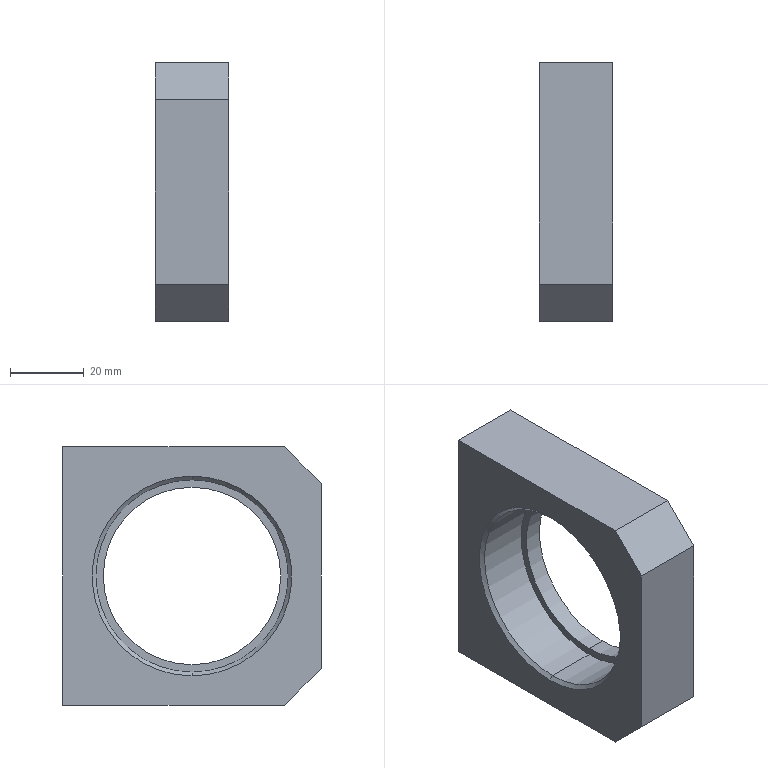Component | SolidWorks | OT-0100-007(BearingHousing)-2 | 1 solid | 23 faces | box 20 x 70 x 70 mm | volume 53530 mm3 | plane 9 | cylinder 8 | cone 6 | commonest cylinder face diameters 6.8 x4 48 x2 52 x2 | material Plain Carbon Steel
build123d program:
from build123d import *

# Parameters (mm, degrees)
SKETCH1_W             = 70
SKETCH1_H             = 70
BOSS_EXTRUDE1_DEPTH   = 20
SKETCH2_R             = 26
CUT_EXTRUDE1_DEPTH    = 15
CUT_EXTRUDE2_REACH    = 81.687
SKETCH3_R             = 24
CHAMFER1_SIZE         = 1
M8_TAPPED_HOLE1_D     = 6.8
M8_TAPPED_HOLE1_DEPTH = 19.75
M8_TAPPED_HOLE1_TIP   = 2.043
CHAMFER2_SIZE         = 10


with BuildPart() as part:
    # Sketch1 → Boss-Extrude1 (new body)
    with BuildSketch(Plane(origin=(0, 0, 0), x_dir=(0, 0, -1), z_dir=(1, 0, 0))):
        with Locations((0, 35)):
            Rectangle(SKETCH1_W, SKETCH1_H)
    extrude(amount=BOSS_EXTRUDE1_DEPTH)

    # Sketch2 → Cut-Extrude1 (cut)
    with BuildSketch(Plane(origin=(20, 0, 0), x_dir=(0, 0, -1), z_dir=(1, 0, 0))):
        with Locations((0, 35)):
            Circle(SKETCH2_R)
    extrude(amount=-CUT_EXTRUDE1_DEPTH, mode=Mode.SUBTRACT)

    # Sketch3 → Cut-Extrude2 (cut, up to next)
    with BuildSketch(Plane(origin=(5, 0, 0), x_dir=(0, 0, -1), z_dir=(1, 0, 0)), mode=Mode.PRIVATE) as cut_extrude2_sk1:
        with Locations((0, 35)):
            Circle(SKETCH3_R)
    cut_extrude2_tool1 = extrude(cut_extrude2_sk1.sketch, amount=-CUT_EXTRUDE2_REACH, mode=Mode.PRIVATE) & part.part
    add(cut_extrude2_tool1.solids().sort_by_distance((5, 35, 0))[0], mode=Mode.SUBTRACT)

    # Chamfer1
    chamfer1_edges = [part.edges().sort_by_distance(p)[0] for p in [
        (20, 35, 26),
    ]]
    chamfer(chamfer1_edges, length=CHAMFER1_SIZE)

    # M8 Tapped Hole1
    with Locations(Plane(origin=(0, 70, 0), x_dir=(1, 0, 0), z_dir=(0, 1, 0))):
        with Locations((10, -27.5), (10, 27.5)):
            Hole(M8_TAPPED_HOLE1_D / 2, depth=M8_TAPPED_HOLE1_DEPTH)
            with Locations((0, 0, -(M8_TAPPED_HOLE1_DEPTH + M8_TAPPED_HOLE1_TIP / 2))):  # 118° drill point
                Cone(0, M8_TAPPED_HOLE1_D / 2, M8_TAPPED_HOLE1_TIP, mode=Mode.SUBTRACT)

    # Chamfer2
    chamfer2_edges = [part.edges().sort_by_distance(p)[0] for p in [
        (10, 0, -35),
        (10, 0, 35),
    ]]
    chamfer(chamfer2_edges, length=CHAMFER2_SIZE)


solid = part.part

# Placed as in the assembly
solid = solid.moved(Location((400, 0, 0), (-180, 0, 180)))
STEP:
#1=COLOUR_RGB('',0.7922,0.8196,0.9333);
#2=FILL_AREA_STYLE_COLOUR('',#1);
#3=FILL_AREA_STYLE('',(#2));
#4=SURFACE_STYLE_FILL_AREA(#3);
#5=SURFACE_SIDE_STYLE('',(#4));
#6=SURFACE_STYLE_USAGE(.BOTH.,#5);
#7=PRESENTATION_STYLE_ASSIGNMENT((#6));
#8=CARTESIAN_POINT('',(15.354,1.978,-0.9488));
#9=VERTEX_POINT('',#8);
#10=CARTESIAN_POINT('',(15.354,1.978,-1.217));
#11=VERTEX_POINT('',#10);
#12=CARTESIAN_POINT('',(15.354,1.978,-1.083));
#13=DIRECTION('',(0.,1.,0.));
#14=DIRECTION('',(0.,0.,-1.));
#15=AXIS2_PLACEMENT_3D('',#12,#13,#14);
#16=CIRCLE('',#15,0.1339);
#17=EDGE_CURVE('',#9,#11,#16,.T.);
#18=ORIENTED_EDGE('',*,*,#17,.F.);
#19=CARTESIAN_POINT('',(15.354,2.756,-0.9488));
#20=VERTEX_POINT('',#19);
#21=CARTESIAN_POINT('',(15.354,2.756,-0.9488));
#22=DIRECTION('',(0.,1.,0.));
#23=VECTOR('',#22,39.37);
#24=LINE('',#21,#23);
#25=EDGE_CURVE('',#9,#20,#24,.T.);
#26=ORIENTED_EDGE('',*,*,#25,.T.);
#27=CARTESIAN_POINT('',(15.354,2.756,-1.217));
#28=VERTEX_POINT('',#27);
#29=CARTESIAN_POINT('',(15.354,2.756,-1.083));
#30=DIRECTION('',(0.,1.,0.));
#31=DIRECTION('',(0.,0.,-1.));
#32=AXIS2_PLACEMENT_3D('',#29,#30,#31);
#33=CIRCLE('',#32,0.1339);
#34=EDGE_CURVE('',#20,#28,#33,.T.);
#35=ORIENTED_EDGE('',*,*,#34,.T.);
#36=CARTESIAN_POINT('',(15.354,2.756,-1.217));
#37=DIRECTION('',(0.,1.,0.));
#38=VECTOR('',#37,39.37);
#39=LINE('',#36,#38);
#40=EDGE_CURVE('',#11,#28,#39,.T.);
#41=ORIENTED_EDGE('',*,*,#40,.F.);
#42=EDGE_LOOP('',(#18,#26,#35,#41));
#43=FACE_OUTER_BOUND('',#42,.T.);
#44=CARTESIAN_POINT('',(15.354,2.756,-1.083));
#45=DIRECTION('',(0.,1.,0.));
#46=DIRECTION('',(0.,0.,-1.));
#47=AXIS2_PLACEMENT_3D('',#44,#45,#46);
#48=CYLINDRICAL_SURFACE('',#47,0.1339);
#49=ADVANCED_FACE('',(#43),#48,.F.);
#50=CARTESIAN_POINT('',(15.354,1.898,-1.083));
#51=VERTEX_POINT('',#50);
#52=CARTESIAN_POINT('',(15.354,1.978,-1.217));
#53=DIRECTION('',(0.,0.515,-0.8572));
#54=VECTOR('',#53,39.37);
#55=LINE('',#52,#54);
#56=EDGE_CURVE('',#51,#11,#55,.T.);
#57=ORIENTED_EDGE('',*,*,#56,.F.);
#58=CARTESIAN_POINT('',(15.354,1.978,-0.9488));
#59=DIRECTION('',(-0.,0.515,0.8572));
#60=VECTOR('',#59,39.37);
#61=LINE('',#58,#60);
#62=EDGE_CURVE('',#51,#9,#61,.T.);
#63=ORIENTED_EDGE('',*,*,#62,.T.);
#64=ORIENTED_EDGE('',*,*,#17,.T.);
#65=EDGE_LOOP('',(#57,#63,#64));
#66=FACE_OUTER_BOUND('',#65,.T.);
#67=CARTESIAN_POINT('',(15.354,1.978,-1.083));
#68=DIRECTION('',(0.,1.,0.));
#69=DIRECTION('',(0.,0.,-1.));
#70=AXIS2_PLACEMENT_3D('',#67,#68,#69);
#71=CONICAL_SURFACE('',#70,0.1339,1.03);
#72=ADVANCED_FACE('',(#66),#71,.F.);
#73=CARTESIAN_POINT('',(15.354,1.978,1.217));
#74=VERTEX_POINT('',#73);
#75=CARTESIAN_POINT('',(15.354,1.978,0.9488));
#76=VERTEX_POINT('',#75);
#77=CARTESIAN_POINT('',(15.354,1.978,1.083));
#78=DIRECTION('',(0.,1.,0.));
#79=DIRECTION('',(0.,0.,-1.));
#80=AXIS2_PLACEMENT_3D('',#77,#78,#79);
#81=CIRCLE('',#80,0.1339);
#82=EDGE_CURVE('',#74,#76,#81,.T.);
#83=ORIENTED_EDGE('',*,*,#82,.F.);
#84=CARTESIAN_POINT('',(15.354,2.756,1.217));
#85=VERTEX_POINT('',#84);
#86=CARTESIAN_POINT('',(15.354,2.756,1.217));
#87=DIRECTION('',(0.,1.,0.));
#88=VECTOR('',#87,39.37);
#89=LINE('',#86,#88);
#90=EDGE_CURVE('',#74,#85,#89,.T.);
#91=ORIENTED_EDGE('',*,*,#90,.T.);
#92=CARTESIAN_POINT('',(15.354,2.756,0.9488));
#93=VERTEX_POINT('',#92);
#94=CARTESIAN_POINT('',(15.354,2.756,1.083));
#95=DIRECTION('',(0.,1.,0.));
#96=DIRECTION('',(0.,0.,-1.));
#97=AXIS2_PLACEMENT_3D('',#94,#95,#96);
#98=CIRCLE('',#97,0.1339);
#99=EDGE_CURVE('',#85,#93,#98,.T.);
#100=ORIENTED_EDGE('',*,*,#99,.T.);
#101=CARTESIAN_POINT('',(15.354,2.756,0.9488));
#102=DIRECTION('',(0.,1.,0.));
#103=VECTOR('',#102,39.37);
#104=LINE('',#101,#103);
#105=EDGE_CURVE('',#76,#93,#104,.T.);
#106=ORIENTED_EDGE('',*,*,#105,.F.);
#107=EDGE_LOOP('',(#83,#91,#100,#106));
#108=FACE_OUTER_BOUND('',#107,.T.);
#109=CARTESIAN_POINT('',(15.354,2.756,1.083));
#110=DIRECTION('',(0.,1.,0.));
#111=DIRECTION('',(0.,0.,-1.));
#112=AXIS2_PLACEMENT_3D('',#109,#110,#111);
#113=CYLINDRICAL_SURFACE('',#112,0.1339);
#114=ADVANCED_FACE('',(#108),#113,.F.);
#115=CARTESIAN_POINT('',(15.354,1.898,1.083));
#116=VERTEX_POINT('',#115);
#117=CARTESIAN_POINT('',(15.354,1.978,0.9488));
#118=DIRECTION('',(0.,0.515,-0.8572));
#119=VECTOR('',#118,39.37);
#120=LINE('',#117,#119);
#121=EDGE_CURVE('',#116,#76,#120,.T.);
#122=ORIENTED_EDGE('',*,*,#121,.F.);
#123=CARTESIAN_POINT('',(15.354,1.978,1.217));
#124=DIRECTION('',(-0.,0.515,0.8572));
#125=VECTOR('',#124,39.37);
#126=LINE('',#123,#125);
#127=EDGE_CURVE('',#116,#74,#126,.T.);
#128=ORIENTED_EDGE('',*,*,#127,.T.);
#129=ORIENTED_EDGE('',*,*,#82,.T.);
#130=EDGE_LOOP('',(#122,#128,#129));
#131=FACE_OUTER_BOUND('',#130,.T.);
#132=CARTESIAN_POINT('',(15.354,1.978,1.083));
#133=DIRECTION('',(0.,1.,0.));
#134=DIRECTION('',(0.,0.,-1.));
#135=AXIS2_PLACEMENT_3D('',#132,#133,#134);
#136=CONICAL_SURFACE('',#135,0.1339,1.03);
#137=ADVANCED_FACE('',(#131),#136,.F.);
#138=CARTESIAN_POINT('',(15.,1.378,-1.024));
#139=VERTEX_POINT('',#138);
#140=CARTESIAN_POINT('',(15.,1.378,1.024));
#141=VERTEX_POINT('',#140);
#142=CARTESIAN_POINT('',(15.,1.378,-0.));
#143=DIRECTION('',(-1.,0.,0.));
#144=DIRECTION('',(0.,0.,-1.));
#145=AXIS2_PLACEMENT_3D('',#142,#143,#144);
#146=CIRCLE('',#145,1.024);
#147=EDGE_CURVE('',#139,#141,#146,.T.);
#148=ORIENTED_EDGE('',*,*,#147,.F.);
#149=CARTESIAN_POINT('',(14.961,1.378,-1.063));
#150=VERTEX_POINT('',#149);
#151=CARTESIAN_POINT('',(15.,1.378,-1.024));
#152=DIRECTION('',(-0.7071,0.,-0.7071));
#153=VECTOR('',#152,39.37);
#154=LINE('',#151,#153);
#155=EDGE_CURVE('',#139,#150,#154,.T.);
#156=ORIENTED_EDGE('',*,*,#155,.T.);
#157=CARTESIAN_POINT('',(14.961,1.378,1.063));
#158=VERTEX_POINT('',#157);
#159=CARTESIAN_POINT('',(14.961,1.378,-0.));
#160=DIRECTION('',(1.,0.,0.));
#161=DIRECTION('',(0.,0.,-1.));
#162=AXIS2_PLACEMENT_3D('',#159,#160,#161);
#163=CIRCLE('',#162,1.063);
#164=EDGE_CURVE('',#158,#150,#163,.T.);
#165=ORIENTED_EDGE('',*,*,#164,.F.);
#166=CARTESIAN_POINT('',(15.,1.378,1.024));
#167=DIRECTION('',(-0.7071,0.,0.7071));
#168=VECTOR('',#167,39.37);
#169=LINE('',#166,#168);
#170=EDGE_CURVE('',#141,#158,#169,.T.);
#171=ORIENTED_EDGE('',*,*,#170,.F.);
#172=EDGE_LOOP('',(#148,#156,#165,#171));
#173=FACE_OUTER_BOUND('',#172,.T.);
#174=CARTESIAN_POINT('',(15.,1.378,-0.));
#175=DIRECTION('',(-1.,0.,0.));
#176=DIRECTION('',(0.,0.,1.));
#177=AXIS2_PLACEMENT_3D('',#174,#175,#176);
#178=CONICAL_SURFACE('',#177,1.024,0.7854);
#179=ADVANCED_FACE('',(#173),#178,.F.);
#180=CARTESIAN_POINT('',(15.748,1.378,-0.9449));
#181=VERTEX_POINT('',#180);
#182=CARTESIAN_POINT('',(15.748,1.378,0.9449));
#183=VERTEX_POINT('',#182);
#184=CARTESIAN_POINT('',(15.748,1.378,-0.));
#185=DIRECTION('',(-1.,0.,0.));
#186=DIRECTION('',(0.,0.,-1.));
#187=AXIS2_PLACEMENT_3D('',#184,#185,#186);
#188=CIRCLE('',#187,0.9449);
#189=EDGE_CURVE('',#181,#183,#188,.T.);
#190=ORIENTED_EDGE('',*,*,#189,.F.);
#191=CARTESIAN_POINT('',(15.551,1.378,-0.9449));
#192=VERTEX_POINT('',#191);
#193=CARTESIAN_POINT('',(15.748,1.378,-0.9449));
#194=DIRECTION('',(-1.,0.,0.));
#195=VECTOR('',#194,39.37);
#196=LINE('',#193,#195);
#197=EDGE_CURVE('',#181,#192,#196,.T.);
#198=ORIENTED_EDGE('',*,*,#197,.T.);
#199=CARTESIAN_POINT('',(15.551,1.378,0.9449));
#200=VERTEX_POINT('',#199);
#201=CARTESIAN_POINT('',(15.551,1.378,-0.));
#202=DIRECTION('',(-1.,0.,0.));
#203=DIRECTION('',(0.,0.,1.));
#204=AXIS2_PLACEMENT_3D('',#201,#202,#203);
#205=CIRCLE('',#204,0.9449);
#206=EDGE_CURVE('',#192,#200,#205,.T.);
#207=ORIENTED_EDGE('',*,*,#206,.T.);
#208=CARTESIAN_POINT('',(15.748,1.378,0.9449));
#209=DIRECTION('',(-1.,0.,0.));
#210=VECTOR('',#209,39.37);
#211=LINE('',#208,#210);
#212=EDGE_CURVE('',#183,#200,#211,.T.);
#213=ORIENTED_EDGE('',*,*,#212,.F.);
#214=EDGE_LOOP('',(#190,#198,#207,#213));
#215=FACE_OUTER_BOUND('',#214,.T.);
#216=CARTESIAN_POINT('',(15.748,1.378,-0.));
#217=DIRECTION('',(-1.,0.,0.));
#218=DIRECTION('',(0.,0.,1.));
#219=AXIS2_PLACEMENT_3D('',#216,#217,#218);
#220=CYLINDRICAL_SURFACE('',#219,0.9449);
#221=ADVANCED_FACE('',(#215),#220,.F.);
#222=CARTESIAN_POINT('',(15.551,1.378,-1.024));
#223=VERTEX_POINT('',#222);
#224=CARTESIAN_POINT('',(15.551,1.378,1.024));
#225=VERTEX_POINT('',#224);
#226=CARTESIAN_POINT('',(15.551,1.378,-0.));
#227=DIRECTION('',(-1.,0.,0.));
#228=DIRECTION('',(0.,0.,1.));
#229=AXIS2_PLACEMENT_3D('',#226,#227,#228);
#230=CIRCLE('',#229,1.024);
#231=EDGE_CURVE('',#223,#225,#230,.T.);
#232=ORIENTED_EDGE('',*,*,#231,.F.);
#233=CARTESIAN_POINT('',(15.551,1.378,-1.024));
#234=DIRECTION('',(-1.,0.,0.));
#235=VECTOR('',#234,39.37);
#236=LINE('',#233,#235);
#237=EDGE_CURVE('',#223,#139,#236,.T.);
#238=ORIENTED_EDGE('',*,*,#237,.T.);
#239=ORIENTED_EDGE('',*,*,#147,.T.);
#240=CARTESIAN_POINT('',(15.551,1.378,1.024));
#241=DIRECTION('',(-1.,0.,0.));
#242=VECTOR('',#241,39.37);
#243=LINE('',#240,#242);
#244=EDGE_CURVE('',#225,#141,#243,.T.);
#245=ORIENTED_EDGE('',*,*,#244,.F.);
#246=EDGE_LOOP('',(#232,#238,#239,#245));
#247=FACE_OUTER_BOUND('',#246,.T.);
#248=CARTESIAN_POINT('',(15.551,1.378,-0.));
#249=DIRECTION('',(-1.,0.,0.));
#250=DIRECTION('',(0.,0.,1.));
#251=AXIS2_PLACEMENT_3D('',#248,#249,#250);
#252=CYLINDRICAL_SURFACE('',#251,1.024);
#253=ADVANCED_FACE('',(#247),#252,.F.);
#254=CARTESIAN_POINT('',(15.748,2.756,-1.378));
#255=VERTEX_POINT('',#254);
#256=CARTESIAN_POINT('',(15.748,0.3937,-1.378));
#257=VERTEX_POINT('',#256);
#258=CARTESIAN_POINT('',(15.748,-0.,-1.378));
#259=DIRECTION('',(0.,-1.,0.));
#260=VECTOR('',#259,39.37);
#261=LINE('',#258,#260);
#262=EDGE_CURVE('',#255,#257,#261,.T.);
#263=ORIENTED_EDGE('',*,*,#262,.T.);
#264=CARTESIAN_POINT('',(14.961,0.3937,-1.378));
#265=VERTEX_POINT('',#264);
#266=CARTESIAN_POINT('',(14.961,0.3937,-1.378));
#267=DIRECTION('',(-1.,0.,0.));
#268=VECTOR('',#267,39.37);
#269=LINE('',#266,#268);
#270=EDGE_CURVE('',#257,#265,#269,.T.);
#271=ORIENTED_EDGE('',*,*,#270,.T.);
#272=CARTESIAN_POINT('',(14.961,2.756,-1.378));
#273=VERTEX_POINT('',#272);
#274=CARTESIAN_POINT('',(14.961,-0.,-1.378));
#275=DIRECTION('',(0.,-1.,0.));
#276=VECTOR('',#275,39.37);
#277=LINE('',#274,#276);
#278=EDGE_CURVE('',#273,#265,#277,.T.);
#279=ORIENTED_EDGE('',*,*,#278,.F.);
#280=CARTESIAN_POINT('',(14.961,2.756,-1.378));
#281=DIRECTION('',(1.,0.,0.));
#282=VECTOR('',#281,39.37);
#283=LINE('',#280,#282);
#284=EDGE_CURVE('',#273,#255,#283,.T.);
#285=ORIENTED_EDGE('',*,*,#284,.T.);
#286=EDGE_LOOP('',(#263,#271,#279,#285));
#287=FACE_OUTER_BOUND('',#286,.T.);
#288=CARTESIAN_POINT('',(14.961,-0.,-1.378));
#289=DIRECTION('',(0.,0.,1.));
#290=DIRECTION('',(1.,0.,0.));
#291=AXIS2_PLACEMENT_3D('',#288,#289,#290);
#292=PLANE('',#291);
#293=ADVANCED_FACE('',(#287),#292,.F.);
#294=CARTESIAN_POINT('',(15.748,-0.,-0.9843));
#295=VERTEX_POINT('',#294);
#296=CARTESIAN_POINT('',(15.748,-0.,0.9843));
#297=VERTEX_POINT('',#296);
#298=CARTESIAN_POINT('',(15.748,-0.,1.378));
#299=DIRECTION('',(0.,0.,1.));
#300=VECTOR('',#299,39.37);
#301=LINE('',#298,#300);
#302=EDGE_CURVE('',#295,#297,#301,.T.);
#303=ORIENTED_EDGE('',*,*,#302,.T.);
#304=CARTESIAN_POINT('',(14.961,-0.,0.9843));
#305=VERTEX_POINT('',#304);
#306=CARTESIAN_POINT('',(14.961,-0.,0.9843));
#307=DIRECTION('',(-1.,0.,0.));
#308=VECTOR('',#307,39.37);
#309=LINE('',#306,#308);
#310=EDGE_CURVE('',#297,#305,#309,.T.);
#311=ORIENTED_EDGE('',*,*,#310,.T.);
#312=CARTESIAN_POINT('',(14.961,-0.,-0.9843));
#313=VERTEX_POINT('',#312);
#314=CARTESIAN_POINT('',(14.961,-0.,1.378));
#315=DIRECTION('',(0.,0.,1.));
#316=VECTOR('',#315,39.37);
#317=LINE('',#314,#316);
#318=EDGE_CURVE('',#313,#305,#317,.T.);
#319=ORIENTED_EDGE('',*,*,#318,.F.);
#320=CARTESIAN_POINT('',(14.961,-0.,-0.9843));
#321=DIRECTION('',(1.,0.,0.));
#322=VECTOR('',#321,39.37);
#323=LINE('',#320,#322);
#324=EDGE_CURVE('',#313,#295,#323,.T.);
#325=ORIENTED_EDGE('',*,*,#324,.T.);
#326=EDGE_LOOP('',(#303,#311,#319,#325));
#327=FACE_OUTER_BOUND('',#326,.T.);
#328=CARTESIAN_POINT('',(14.961,-0.,1.378));
#329=DIRECTION('',(0.,1.,0.));
#330=DIRECTION('',(0.,0.,-1.));
#331=AXIS2_PLACEMENT_3D('',#328,#329,#330);
#332=PLANE('',#331);
#333=ADVANCED_FACE('',(#327),#332,.F.);
#334=CARTESIAN_POINT('',(14.961,0.3937,1.378));
#335=VERTEX_POINT('',#334);
#336=CARTESIAN_POINT('',(14.961,2.756,1.378));
#337=VERTEX_POINT('',#336);
#338=CARTESIAN_POINT('',(14.961,-0.,1.378));
#339=DIRECTION('',(0.,1.,0.));
#340=VECTOR('',#339,39.37);
#341=LINE('',#338,#340);
#342=EDGE_CURVE('',#335,#337,#341,.T.);
#343=ORIENTED_EDGE('',*,*,#342,.F.);
#344=CARTESIAN_POINT('',(15.748,0.3937,1.378));
#345=VERTEX_POINT('',#344);
#346=CARTESIAN_POINT('',(14.961,0.3937,1.378));
#347=DIRECTION('',(1.,0.,0.));
#348=VECTOR('',#347,39.37);
#349=LINE('',#346,#348);
#350=EDGE_CURVE('',#335,#345,#349,.T.);
#351=ORIENTED_EDGE('',*,*,#350,.T.);
#352=CARTESIAN_POINT('',(15.748,2.756,1.378));
#353=VERTEX_POINT('',#352);
#354=CARTESIAN_POINT('',(15.748,-0.,1.378));
#355=DIRECTION('',(0.,1.,0.));
#356=VECTOR('',#355,39.37);
#357=LINE('',#354,#356);
#358=EDGE_CURVE('',#345,#353,#357,.T.);
#359=ORIENTED_EDGE('',*,*,#358,.T.);
#360=CARTESIAN_POINT('',(14.961,2.756,1.378));
#361=DIRECTION('',(1.,0.,0.));
#362=VECTOR('',#361,39.37);
#363=LINE('',#360,#362);
#364=EDGE_CURVE('',#337,#353,#363,.T.);
#365=ORIENTED_EDGE('',*,*,#364,.F.);
#366=EDGE_LOOP('',(#343,#351,#359,#365));
#367=FACE_OUTER_BOUND('',#366,.T.);
#368=CARTESIAN_POINT('',(14.961,-0.,1.378));
#369=DIRECTION('',(0.,0.,-1.));
#370=DIRECTION('',(-1.,0.,0.));
#371=AXIS2_PLACEMENT_3D('',#368,#369,#370);
#372=PLANE('',#371);
#373=ADVANCED_FACE('',(#367),#372,.F.);
#374=CARTESIAN_POINT('',(15.354,2.756,-1.083));
#375=DIRECTION('',(0.,1.,0.));
#376=DIRECTION('',(0.,0.,-1.));
#377=AXIS2_PLACEMENT_3D('',#374,#375,#376);
#378=CIRCLE('',#377,0.1339);
#379=EDGE_CURVE('',#28,#20,#378,.T.);
#380=ORIENTED_EDGE('',*,*,#379,.F.);
#381=ORIENTED_EDGE('',*,*,#34,.F.);
#382=EDGE_LOOP('',(#380,#381));
#383=FACE_BOUND('',#382,.T.);
#384=CARTESIAN_POINT('',(15.354,2.756,1.083));
#385=DIRECTION('',(0.,1.,0.));
#386=DIRECTION('',(0.,0.,-1.));
#387=AXIS2_PLACEMENT_3D('',#384,#385,#386);
#388=CIRCLE('',#387,0.1339);
#389=EDGE_CURVE('',#93,#85,#388,.T.);
#390=ORIENTED_EDGE('',*,*,#389,.F.);
#391=ORIENTED_EDGE('',*,*,#99,.F.);
#392=EDGE_LOOP('',(#390,#391));
#393=FACE_BOUND('',#392,.T.);
#394=CARTESIAN_POINT('',(15.748,2.756,-1.378));
#395=DIRECTION('',(0.,0.,-1.));
#396=VECTOR('',#395,39.37);
#397=LINE('',#394,#396);
#398=EDGE_CURVE('',#353,#255,#397,.T.);
#399=ORIENTED_EDGE('',*,*,#398,.T.);
#400=ORIENTED_EDGE('',*,*,#284,.F.);
#401=CARTESIAN_POINT('',(14.961,2.756,-1.378));
#402=DIRECTION('',(0.,0.,-1.));
#403=VECTOR('',#402,39.37);
#404=LINE('',#401,#403);
#405=EDGE_CURVE('',#337,#273,#404,.T.);
#406=ORIENTED_EDGE('',*,*,#405,.F.);
#407=ORIENTED_EDGE('',*,*,#364,.T.);
#408=EDGE_LOOP('',(#399,#400,#406,#407));
#409=FACE_OUTER_BOUND('',#408,.T.);
#410=CARTESIAN_POINT('',(14.961,2.756,-1.378));
#411=DIRECTION('',(0.,-1.,0.));
#412=DIRECTION('',(0.,0.,1.));
#413=AXIS2_PLACEMENT_3D('',#410,#411,#412);
#414=PLANE('',#413);
#415=ADVANCED_FACE('',(#383,#393,#409),#414,.F.);
#416=ORIENTED_EDGE('',*,*,#164,.T.);
#417=CARTESIAN_POINT('',(14.961,1.378,-0.));
#418=DIRECTION('',(1.,0.,0.));
#419=DIRECTION('',(0.,0.,-1.));
#420=AXIS2_PLACEMENT_3D('',#417,#418,#419);
#421=CIRCLE('',#420,1.063);
#422=EDGE_CURVE('',#150,#158,#421,.T.);
#423=ORIENTED_EDGE('',*,*,#422,.T.);
#424=EDGE_LOOP('',(#416,#423));
#425=FACE_BOUND('',#424,.T.);
#426=ORIENTED_EDGE('',*,*,#318,.T.);
#427=CARTESIAN_POINT('',(14.961,0.3937,1.378));
#428=DIRECTION('',(0.,0.7071,0.7071));
#429=VECTOR('',#428,39.37);
#430=LINE('',#427,#429);
#431=EDGE_CURVE('',#305,#335,#430,.T.);
#432=ORIENTED_EDGE('',*,*,#431,.T.);
#433=ORIENTED_EDGE('',*,*,#342,.T.);
#434=ORIENTED_EDGE('',*,*,#405,.T.);
#435=ORIENTED_EDGE('',*,*,#278,.T.);
#436=CARTESIAN_POINT('',(14.961,-0.,-0.9843));
#437=DIRECTION('',(0.,-0.7071,0.7071));
#438=VECTOR('',#437,39.37);
#439=LINE('',#436,#438);
#440=EDGE_CURVE('',#265,#313,#439,.T.);
#441=ORIENTED_EDGE('',*,*,#440,.T.);
#442=EDGE_LOOP('',(#426,#432,#433,#434,#435,#441));
#443=FACE_OUTER_BOUND('',#442,.T.);
#444=CARTESIAN_POINT('',(14.961,-0.,-0.));
#445=DIRECTION('',(1.,0.,0.));
#446=DIRECTION('',(0.,0.,-1.));
#447=AXIS2_PLACEMENT_3D('',#444,#445,#446);
#448=PLANE('',#447);
#449=ADVANCED_FACE('',(#425,#443),#448,.F.);
#450=CARTESIAN_POINT('',(15.748,1.378,-0.));
#451=DIRECTION('',(-1.,0.,0.));
#452=DIRECTION('',(0.,0.,-1.));
#453=AXIS2_PLACEMENT_3D('',#450,#451,#452);
#454=CIRCLE('',#453,0.9449);
#455=EDGE_CURVE('',#183,#181,#454,.T.);
#456=ORIENTED_EDGE('',*,*,#455,.T.);
#457=ORIENTED_EDGE('',*,*,#189,.T.);
#458=EDGE_LOOP('',(#456,#457));
#459=FACE_BOUND('',#458,.T.);
#460=ORIENTED_EDGE('',*,*,#358,.F.);
#461=CARTESIAN_POINT('',(15.748,-0.4921,0.4921));
#462=DIRECTION('',(0.,-0.7071,-0.7071));
#463=VECTOR('',#462,39.37);
#464=LINE('',#461,#463);
#465=EDGE_CURVE('',#345,#297,#464,.T.);
#466=ORIENTED_EDGE('',*,*,#465,.T.);
#467=ORIENTED_EDGE('',*,*,#302,.F.);
#468=CARTESIAN_POINT('',(15.748,-0.4921,-0.4921));
#469=DIRECTION('',(0.,0.7071,-0.7071));
#470=VECTOR('',#469,39.37);
#471=LINE('',#468,#470);
#472=EDGE_CURVE('',#295,#257,#471,.T.);
#473=ORIENTED_EDGE('',*,*,#472,.T.);
#474=ORIENTED_EDGE('',*,*,#262,.F.);
#475=ORIENTED_EDGE('',*,*,#398,.F.);
#476=EDGE_LOOP('',(#460,#466,#467,#473,#474,#475));
#477=FACE_OUTER_BOUND('',#476,.T.);
#478=CARTESIAN_POINT('',(15.748,-0.,-0.));
#479=DIRECTION('',(1.,0.,0.));
#480=DIRECTION('',(0.,0.,-1.));
#481=AXIS2_PLACEMENT_3D('',#478,#479,#480);
#482=PLANE('',#481);
#483=ADVANCED_FACE('',(#459,#477),#482,.T.);
#484=ORIENTED_EDGE('',*,*,#237,.F.);
#485=CARTESIAN_POINT('',(15.551,1.378,-0.));
#486=DIRECTION('',(-1.,0.,0.));
#487=DIRECTION('',(0.,0.,1.));
#488=AXIS2_PLACEMENT_3D('',#485,#486,#487);
#489=CIRCLE('',#488,1.024);
#490=EDGE_CURVE('',#225,#223,#489,.T.);
#491=ORIENTED_EDGE('',*,*,#490,.F.);
#492=ORIENTED_EDGE('',*,*,#244,.T.);
#493=CARTESIAN_POINT('',(15.,1.378,-0.));
#494=DIRECTION('',(-1.,0.,0.));
#495=DIRECTION('',(0.,0.,-1.));
#496=AXIS2_PLACEMENT_3D('',#493,#494,#495);
#497=CIRCLE('',#496,1.024);
#498=EDGE_CURVE('',#141,#139,#497,.T.);
#499=ORIENTED_EDGE('',*,*,#498,.T.);
#500=EDGE_LOOP('',(#484,#491,#492,#499));
#501=FACE_OUTER_BOUND('',#500,.T.);
#502=CARTESIAN_POINT('',(15.551,1.378,-0.));
#503=DIRECTION('',(-1.,0.,0.));
#504=DIRECTION('',(0.,0.,1.));
#505=AXIS2_PLACEMENT_3D('',#502,#503,#504);
#506=CYLINDRICAL_SURFACE('',#505,1.024);
#507=ADVANCED_FACE('',(#501),#506,.F.);
#508=CARTESIAN_POINT('',(15.551,1.378,-0.));
#509=DIRECTION('',(-1.,0.,0.));
#510=DIRECTION('',(0.,0.,1.));
#511=AXIS2_PLACEMENT_3D('',#508,#509,#510);
#512=CIRCLE('',#511,0.9449);
#513=EDGE_CURVE('',#200,#192,#512,.T.);
#514=ORIENTED_EDGE('',*,*,#513,.F.);
#515=ORIENTED_EDGE('',*,*,#206,.F.);
#516=EDGE_LOOP('',(#514,#515));
#517=FACE_BOUND('',#516,.T.);
#518=ORIENTED_EDGE('',*,*,#490,.T.);
#519=ORIENTED_EDGE('',*,*,#231,.T.);
#520=EDGE_LOOP('',(#518,#519));
#521=FACE_OUTER_BOUND('',#520,.T.);
#522=CARTESIAN_POINT('',(15.551,1.378,-0.));
#523=DIRECTION('',(-1.,0.,0.));
#524=DIRECTION('',(0.,0.,1.));
#525=AXIS2_PLACEMENT_3D('',#522,#523,#524);
#526=PLANE('',#525);
#527=ADVANCED_FACE('',(#517,#521),#526,.T.);
#528=ORIENTED_EDGE('',*,*,#197,.F.);
#529=ORIENTED_EDGE('',*,*,#455,.F.);
#530=ORIENTED_EDGE('',*,*,#212,.T.);
#531=ORIENTED_EDGE('',*,*,#513,.T.);
#532=EDGE_LOOP('',(#528,#529,#530,#531));
#533=FACE_OUTER_BOUND('',#532,.T.);
#534=CARTESIAN_POINT('',(15.748,1.378,-0.));
#535=DIRECTION('',(-1.,0.,0.));
#536=DIRECTION('',(0.,0.,1.));
#537=AXIS2_PLACEMENT_3D('',#534,#535,#536);
#538=CYLINDRICAL_SURFACE('',#537,0.9449);
#539=ADVANCED_FACE('',(#533),#538,.F.);
#540=ORIENTED_EDGE('',*,*,#155,.F.);
#541=ORIENTED_EDGE('',*,*,#498,.F.);
#542=ORIENTED_EDGE('',*,*,#170,.T.);
#543=ORIENTED_EDGE('',*,*,#422,.F.);
#544=EDGE_LOOP('',(#540,#541,#542,#543));
#545=FACE_OUTER_BOUND('',#544,.T.);
#546=CARTESIAN_POINT('',(15.,1.378,-0.));
#547=DIRECTION('',(-1.,0.,0.));
#548=DIRECTION('',(0.,0.,1.));
#549=AXIS2_PLACEMENT_3D('',#546,#547,#548);
#550=CONICAL_SURFACE('',#549,1.024,0.7854);
#551=ADVANCED_FACE('',(#545),#550,.F.);
#552=ORIENTED_EDGE('',*,*,#127,.F.);
#553=ORIENTED_EDGE('',*,*,#121,.T.);
#554=CARTESIAN_POINT('',(15.354,1.978,1.083));
#555=DIRECTION('',(0.,1.,0.));
#556=DIRECTION('',(0.,0.,-1.));
#557=AXIS2_PLACEMENT_3D('',#554,#555,#556);
#558=CIRCLE('',#557,0.1339);
#559=EDGE_CURVE('',#76,#74,#558,.T.);
#560=ORIENTED_EDGE('',*,*,#559,.T.);
#561=EDGE_LOOP('',(#552,#553,#560));
#562=FACE_OUTER_BOUND('',#561,.T.);
#563=CARTESIAN_POINT('',(15.354,1.978,1.083));
#564=DIRECTION('',(0.,1.,0.));
#565=DIRECTION('',(0.,0.,-1.));
#566=AXIS2_PLACEMENT_3D('',#563,#564,#565);
#567=CONICAL_SURFACE('',#566,0.1339,1.03);
#568=ADVANCED_FACE('',(#562),#567,.F.);
#569=ORIENTED_EDGE('',*,*,#90,.F.);
#570=ORIENTED_EDGE('',*,*,#559,.F.);
#571=ORIENTED_EDGE('',*,*,#105,.T.);
#572=ORIENTED_EDGE('',*,*,#389,.T.);
#573=EDGE_LOOP('',(#569,#570,#571,#572));
#574=FACE_OUTER_BOUND('',#573,.T.);
#575=CARTESIAN_POINT('',(15.354,2.756,1.083));
#576=DIRECTION('',(0.,1.,0.));
#577=DIRECTION('',(0.,0.,-1.));
#578=AXIS2_PLACEMENT_3D('',#575,#576,#577);
#579=CYLINDRICAL_SURFACE('',#578,0.1339);
#580=ADVANCED_FACE('',(#574),#579,.F.);
#581=ORIENTED_EDGE('',*,*,#62,.F.);
#582=ORIENTED_EDGE('',*,*,#56,.T.);
#583=CARTESIAN_POINT('',(15.354,1.978,-1.083));
#584=DIRECTION('',(0.,1.,0.));
#585=DIRECTION('',(0.,0.,-1.));
#586=AXIS2_PLACEMENT_3D('',#583,#584,#585);
#587=CIRCLE('',#586,0.1339);
#588=EDGE_CURVE('',#11,#9,#587,.T.);
#589=ORIENTED_EDGE('',*,*,#588,.T.);
#590=EDGE_LOOP('',(#581,#582,#589));
#591=FACE_OUTER_BOUND('',#590,.T.);
#592=CARTESIAN_POINT('',(15.354,1.978,-1.083));
#593=DIRECTION('',(0.,1.,0.));
#594=DIRECTION('',(0.,0.,-1.));
#595=AXIS2_PLACEMENT_3D('',#592,#593,#594);
#596=CONICAL_SURFACE('',#595,0.1339,1.03);
#597=ADVANCED_FACE('',(#591),#596,.F.);
#598=ORIENTED_EDGE('',*,*,#25,.F.);
#599=ORIENTED_EDGE('',*,*,#588,.F.);
#600=ORIENTED_EDGE('',*,*,#40,.T.);
#601=ORIENTED_EDGE('',*,*,#379,.T.);
#602=EDGE_LOOP('',(#598,#599,#600,#601));
#603=FACE_OUTER_BOUND('',#602,.T.);
#604=CARTESIAN_POINT('',(15.354,2.756,-1.083));
#605=DIRECTION('',(0.,1.,0.));
#606=DIRECTION('',(0.,0.,-1.));
#607=AXIS2_PLACEMENT_3D('',#604,#605,#606);
#608=CYLINDRICAL_SURFACE('',#607,0.1339);
#609=ADVANCED_FACE('',(#603),#608,.F.);
#610=ORIENTED_EDGE('',*,*,#431,.F.);
#611=ORIENTED_EDGE('',*,*,#310,.F.);
#612=ORIENTED_EDGE('',*,*,#465,.F.);
#613=ORIENTED_EDGE('',*,*,#350,.F.);
#614=EDGE_LOOP('',(#610,#611,#612,#613));
#615=FACE_OUTER_BOUND('',#614,.T.);
#616=CARTESIAN_POINT('',(14.961,0.3937,1.378));
#617=DIRECTION('',(0.,0.7071,-0.7071));
#618=DIRECTION('',(1.,0.,0.));
#619=AXIS2_PLACEMENT_3D('',#616,#617,#618);
#620=PLANE('',#619);
#621=ADVANCED_FACE('',(#615),#620,.F.);
#622=ORIENTED_EDGE('',*,*,#440,.F.);
#623=ORIENTED_EDGE('',*,*,#270,.F.);
#624=ORIENTED_EDGE('',*,*,#472,.F.);
#625=ORIENTED_EDGE('',*,*,#324,.F.);
#626=EDGE_LOOP('',(#622,#623,#624,#625));
#627=FACE_OUTER_BOUND('',#626,.T.);
#628=CARTESIAN_POINT('',(14.961,-0.,-0.9843));
#629=DIRECTION('',(0.,0.7071,0.7071));
#630=DIRECTION('',(1.,0.,0.));
#631=AXIS2_PLACEMENT_3D('',#628,#629,#630);
#632=PLANE('',#631);
#633=ADVANCED_FACE('',(#627),#632,.F.);
#634=CLOSED_SHELL('',(#49,#72,#114,#137,#179,#221,#253,#293,#333,#373,#415,#449,#483,#507,#527,#539,#551,#568,#580,#597,#609,#621,#633));
#635=MANIFOLD_SOLID_BREP('',#634);
#636=STYLED_ITEM('',(#7),#635);
#637=PRESENTATION_LAYER_ASSIGNMENT('','',(#636));
#638=(LENGTH_UNIT()NAMED_UNIT(*)SI_UNIT($,.METRE.));
#639=LENGTH_MEASURE_WITH_UNIT(LENGTH_MEASURE(0.0254),#638);
#640=DIMENSIONAL_EXPONENTS(1.,0.,0.,0.,0.,0.,0.);
#641=(CONVERSION_BASED_UNIT('',#639)LENGTH_UNIT()NAMED_UNIT(#640));
#642=UNCERTAINTY_MEASURE_WITH_UNIT(LENGTH_MEASURE(0.00001),#641,'','');
#643=(NAMED_UNIT(*)PLANE_ANGLE_UNIT()SI_UNIT($,.RADIAN.));
#644=(NAMED_UNIT(*)SI_UNIT($,.STERADIAN.)SOLID_ANGLE_UNIT());
#645=(GEOMETRIC_REPRESENTATION_CONTEXT(3)GLOBAL_UNCERTAINTY_ASSIGNED_CONTEXT((#642))GLOBAL_UNIT_ASSIGNED_CONTEXT((#641,#643,#644))REPRESENTATION_CONTEXT('',''));
#646=MECHANICAL_DESIGN_GEOMETRIC_PRESENTATION_REPRESENTATION('',(#636),#645);
#647=CARTESIAN_POINT('',(0.,0.,0.));
#648=DIRECTION('',(0.,0.,1.));
#649=DIRECTION('',(1.,0.,0.));
#650=AXIS2_PLACEMENT_3D('',#647,#648,#649);
#651=(LENGTH_UNIT()NAMED_UNIT(*)SI_UNIT($,.METRE.));
#652=LENGTH_MEASURE_WITH_UNIT(LENGTH_MEASURE(0.0254),#651);
#653=DIMENSIONAL_EXPONENTS(1.,0.,0.,0.,0.,0.,0.);
#654=(CONVERSION_BASED_UNIT('',#652)LENGTH_UNIT()NAMED_UNIT(#653));
#655=UNCERTAINTY_MEASURE_WITH_UNIT(LENGTH_MEASURE(0.00001),#654,'','');
#656=(NAMED_UNIT(*)PLANE_ANGLE_UNIT()SI_UNIT($,.RADIAN.));
#657=(NAMED_UNIT(*)SI_UNIT($,.STERADIAN.)SOLID_ANGLE_UNIT());
#658=(GEOMETRIC_REPRESENTATION_CONTEXT(3)GLOBAL_UNCERTAINTY_ASSIGNED_CONTEXT((#655))GLOBAL_UNIT_ASSIGNED_CONTEXT((#654,#656,#657))REPRESENTATION_CONTEXT('',''));
#659=ADVANCED_BREP_SHAPE_REPRESENTATION('',(#635,#650),#658);